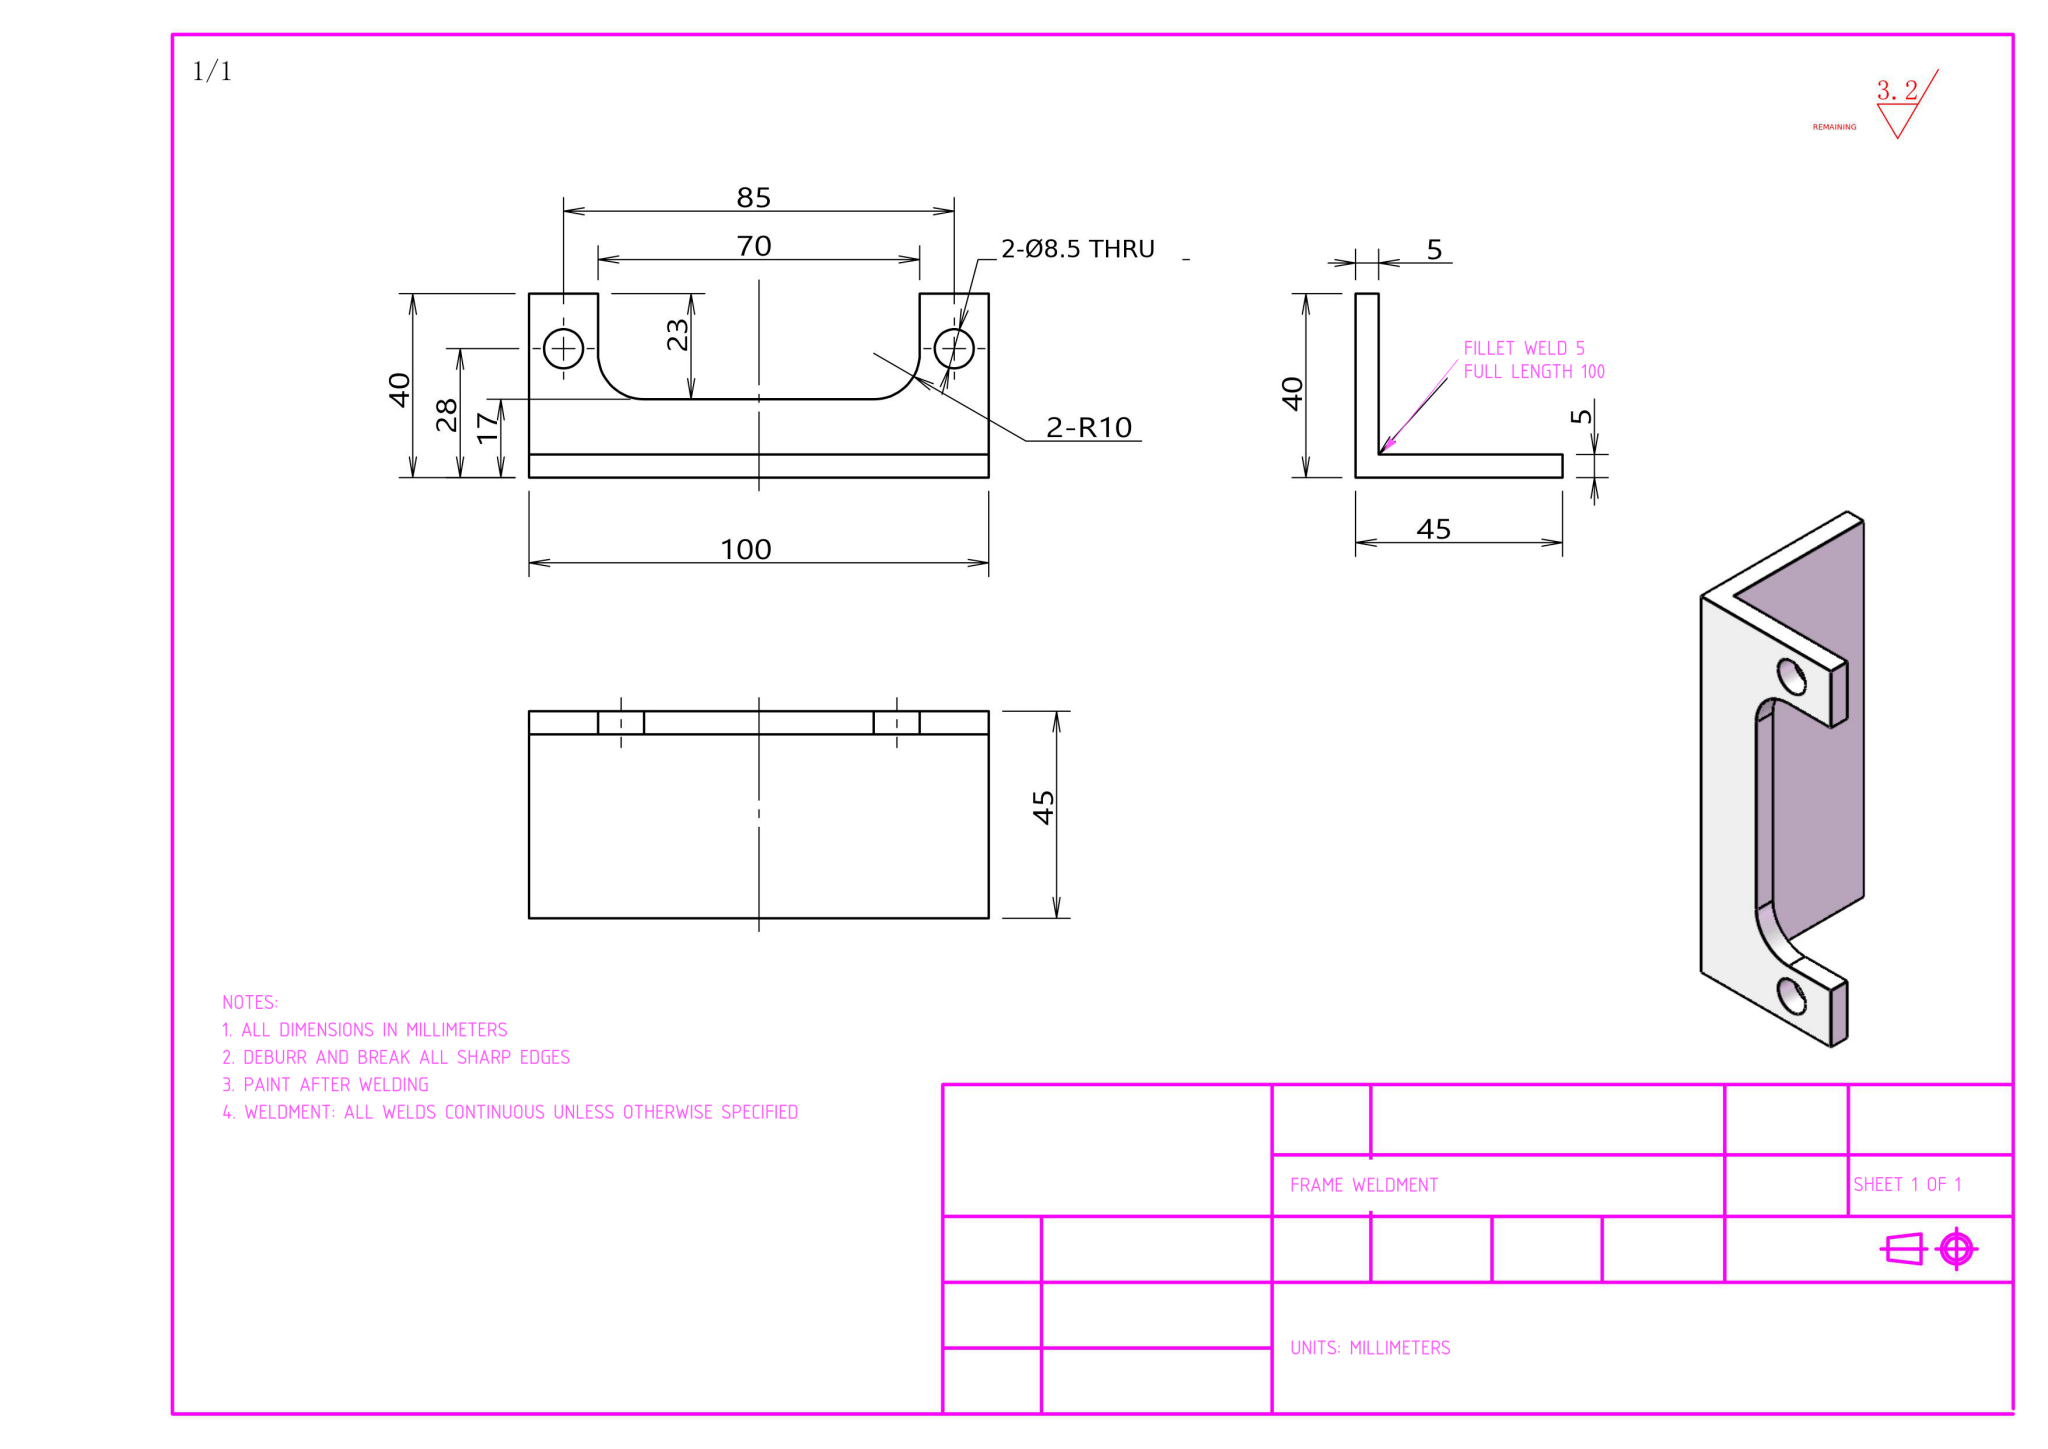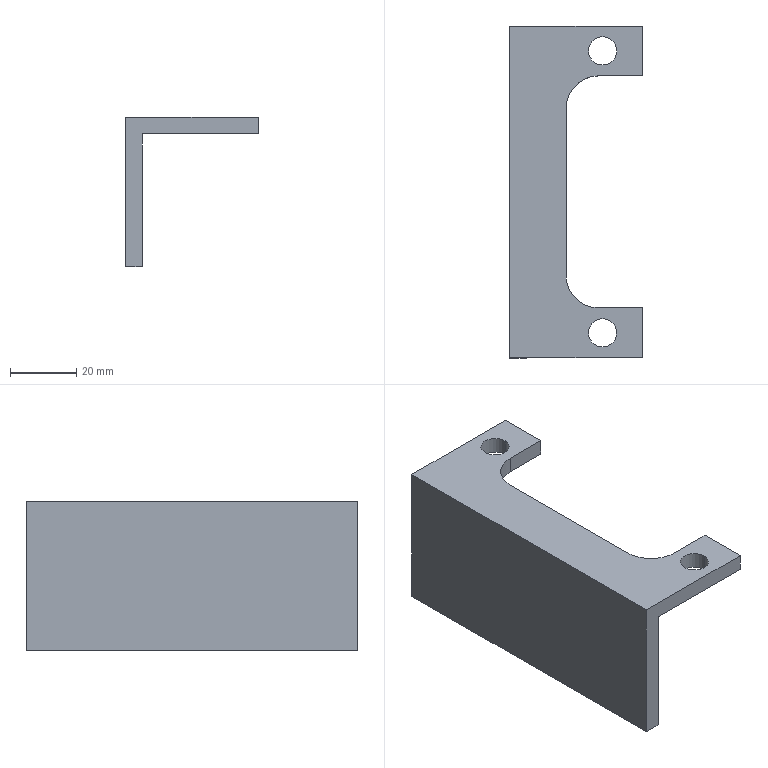Part | NX | mm | 1 solid | 18 faces | box 40 x 100 x 45 mm | volume 31597 mm3 | plane 12 | cylinder 6 | commonest cylinder face diameters 8.5 x4 20 x2
STEP:
#1=COLOUR_RGB('',1.,1.,1.);
#2=FILL_AREA_STYLE_COLOUR('',#1);
#3=FILL_AREA_STYLE('',(#2));
#4=SURFACE_STYLE_FILL_AREA(#3);
#5=SURFACE_SIDE_STYLE('',(#4));
#6=SURFACE_STYLE_USAGE(.BOTH.,#5);
#7=PRESENTATION_STYLE_ASSIGNMENT((#6));
#8=CARTESIAN_POINT('',(32.25,42.5,0.));
#9=VERTEX_POINT('',#8);
#10=CARTESIAN_POINT('',(23.75,42.5,0.));
#11=VERTEX_POINT('',#10);
#12=CARTESIAN_POINT('',(28.,42.5,0.));
#13=DIRECTION('',(0.,0.,-1.));
#14=DIRECTION('',(-1.,0.,0.));
#15=AXIS2_PLACEMENT_3D('',#12,#13,#14);
#16=CIRCLE('',#15,4.25);
#17=EDGE_CURVE('',#9,#11,#16,.T.);
#18=ORIENTED_EDGE('',*,*,#17,.F.);
#19=CARTESIAN_POINT('',(32.25,42.5,-5.));
#20=VERTEX_POINT('',#19);
#21=CARTESIAN_POINT('',(32.25,42.5,-5.));
#22=DIRECTION('',(0.,0.,-1.));
#23=VECTOR('',#22,1000.);
#24=LINE('',#21,#23);
#25=EDGE_CURVE('',#9,#20,#24,.T.);
#26=ORIENTED_EDGE('',*,*,#25,.T.);
#27=CARTESIAN_POINT('',(23.75,42.5,-5.));
#28=VERTEX_POINT('',#27);
#29=CARTESIAN_POINT('',(28.,42.5,-5.));
#30=DIRECTION('',(0.,0.,-1.));
#31=DIRECTION('',(-1.,0.,0.));
#32=AXIS2_PLACEMENT_3D('',#29,#30,#31);
#33=CIRCLE('',#32,4.25);
#34=EDGE_CURVE('',#20,#28,#33,.T.);
#35=ORIENTED_EDGE('',*,*,#34,.T.);
#36=CARTESIAN_POINT('',(23.75,42.5,-5.));
#37=DIRECTION('',(0.,0.,-1.));
#38=VECTOR('',#37,1000.);
#39=LINE('',#36,#38);
#40=EDGE_CURVE('',#11,#28,#39,.T.);
#41=ORIENTED_EDGE('',*,*,#40,.F.);
#42=EDGE_LOOP('',(#18,#26,#35,#41));
#43=FACE_OUTER_BOUND('',#42,.T.);
#44=CARTESIAN_POINT('',(28.,42.5,-5.));
#45=DIRECTION('',(0.,0.,-1.));
#46=DIRECTION('',(-1.,0.,0.));
#47=AXIS2_PLACEMENT_3D('',#44,#45,#46);
#48=CYLINDRICAL_SURFACE('',#47,4.25);
#49=ADVANCED_FACE('',(#43),#48,.F.);
#50=CARTESIAN_POINT('',(32.25,-42.5,0.));
#51=VERTEX_POINT('',#50);
#52=CARTESIAN_POINT('',(23.75,-42.5,0.));
#53=VERTEX_POINT('',#52);
#54=CARTESIAN_POINT('',(28.,-42.5,0.));
#55=DIRECTION('',(0.,0.,-1.));
#56=DIRECTION('',(-1.,0.,0.));
#57=AXIS2_PLACEMENT_3D('',#54,#55,#56);
#58=CIRCLE('',#57,4.25);
#59=EDGE_CURVE('',#51,#53,#58,.T.);
#60=ORIENTED_EDGE('',*,*,#59,.F.);
#61=CARTESIAN_POINT('',(32.25,-42.5,-5.));
#62=VERTEX_POINT('',#61);
#63=CARTESIAN_POINT('',(32.25,-42.5,-5.));
#64=DIRECTION('',(0.,0.,-1.));
#65=VECTOR('',#64,1000.);
#66=LINE('',#63,#65);
#67=EDGE_CURVE('',#51,#62,#66,.T.);
#68=ORIENTED_EDGE('',*,*,#67,.T.);
#69=CARTESIAN_POINT('',(23.75,-42.5,-5.));
#70=VERTEX_POINT('',#69);
#71=CARTESIAN_POINT('',(28.,-42.5,-5.));
#72=DIRECTION('',(0.,0.,-1.));
#73=DIRECTION('',(-1.,0.,0.));
#74=AXIS2_PLACEMENT_3D('',#71,#72,#73);
#75=CIRCLE('',#74,4.25);
#76=EDGE_CURVE('',#62,#70,#75,.T.);
#77=ORIENTED_EDGE('',*,*,#76,.T.);
#78=CARTESIAN_POINT('',(23.75,-42.5,-5.));
#79=DIRECTION('',(0.,0.,-1.));
#80=VECTOR('',#79,1000.);
#81=LINE('',#78,#80);
#82=EDGE_CURVE('',#53,#70,#81,.T.);
#83=ORIENTED_EDGE('',*,*,#82,.F.);
#84=EDGE_LOOP('',(#60,#68,#77,#83));
#85=FACE_OUTER_BOUND('',#84,.T.);
#86=CARTESIAN_POINT('',(28.,-42.5,-5.));
#87=DIRECTION('',(0.,0.,-1.));
#88=DIRECTION('',(-1.,0.,0.));
#89=AXIS2_PLACEMENT_3D('',#86,#87,#88);
#90=CYLINDRICAL_SURFACE('',#89,4.25);
#91=ADVANCED_FACE('',(#85),#90,.F.);
#92=CARTESIAN_POINT('',(40.,50.,-5.));
#93=VERTEX_POINT('',#92);
#94=CARTESIAN_POINT('',(40.,35.,-5.));
#95=VERTEX_POINT('',#94);
#96=CARTESIAN_POINT('',(40.,50.,-5.));
#97=DIRECTION('',(0.,-1.,0.));
#98=VECTOR('',#97,1000.);
#99=LINE('',#96,#98);
#100=EDGE_CURVE('',#93,#95,#99,.T.);
#101=ORIENTED_EDGE('',*,*,#100,.T.);
#102=CARTESIAN_POINT('',(27.,35.,-5.));
#103=VERTEX_POINT('',#102);
#104=CARTESIAN_POINT('',(40.,35.,-5.));
#105=DIRECTION('',(1.,-0.,-0.));
#106=VECTOR('',#105,1000.);
#107=LINE('',#104,#106);
#108=EDGE_CURVE('',#103,#95,#107,.T.);
#109=ORIENTED_EDGE('',*,*,#108,.F.);
#110=CARTESIAN_POINT('',(17.,25.,-5.));
#111=VERTEX_POINT('',#110);
#112=CARTESIAN_POINT('',(27.,25.,-5.));
#113=DIRECTION('',(0.,0.,1.));
#114=DIRECTION('',(1.,0.,-0.));
#115=AXIS2_PLACEMENT_3D('',#112,#113,#114);
#116=CIRCLE('',#115,10.);
#117=EDGE_CURVE('',#103,#111,#116,.T.);
#118=ORIENTED_EDGE('',*,*,#117,.T.);
#119=CARTESIAN_POINT('',(17.,-25.,-5.));
#120=VERTEX_POINT('',#119);
#121=CARTESIAN_POINT('',(17.,35.,-5.));
#122=DIRECTION('',(0.,1.,0.));
#123=VECTOR('',#122,1000.);
#124=LINE('',#121,#123);
#125=EDGE_CURVE('',#120,#111,#124,.T.);
#126=ORIENTED_EDGE('',*,*,#125,.F.);
#127=CARTESIAN_POINT('',(27.,-35.,-5.));
#128=VERTEX_POINT('',#127);
#129=CARTESIAN_POINT('',(27.,-25.,-5.));
#130=DIRECTION('',(0.,0.,1.));
#131=DIRECTION('',(1.,0.,-0.));
#132=AXIS2_PLACEMENT_3D('',#129,#130,#131);
#133=CIRCLE('',#132,10.);
#134=EDGE_CURVE('',#120,#128,#133,.T.);
#135=ORIENTED_EDGE('',*,*,#134,.T.);
#136=CARTESIAN_POINT('',(40.,-35.,-5.));
#137=VERTEX_POINT('',#136);
#138=CARTESIAN_POINT('',(40.,-35.,-5.));
#139=DIRECTION('',(-1.,0.,0.));
#140=VECTOR('',#139,1000.);
#141=LINE('',#138,#140);
#142=EDGE_CURVE('',#137,#128,#141,.T.);
#143=ORIENTED_EDGE('',*,*,#142,.F.);
#144=CARTESIAN_POINT('',(40.,-50.,-5.));
#145=VERTEX_POINT('',#144);
#146=CARTESIAN_POINT('',(40.,50.,-5.));
#147=DIRECTION('',(0.,-1.,0.));
#148=VECTOR('',#147,1000.);
#149=LINE('',#146,#148);
#150=EDGE_CURVE('',#137,#145,#149,.T.);
#151=ORIENTED_EDGE('',*,*,#150,.T.);
#152=CARTESIAN_POINT('',(5.,-50.,-5.));
#153=VERTEX_POINT('',#152);
#154=CARTESIAN_POINT('',(40.,-50.,-5.));
#155=DIRECTION('',(-1.,0.,0.));
#156=VECTOR('',#155,1000.);
#157=LINE('',#154,#156);
#158=EDGE_CURVE('',#145,#153,#157,.T.);
#159=ORIENTED_EDGE('',*,*,#158,.T.);
#160=CARTESIAN_POINT('',(5.,50.,-5.));
#161=VERTEX_POINT('',#160);
#162=CARTESIAN_POINT('',(5.,50.,-5.));
#163=DIRECTION('',(0.,-1.,0.));
#164=VECTOR('',#163,1000.);
#165=LINE('',#162,#164);
#166=EDGE_CURVE('',#161,#153,#165,.T.);
#167=ORIENTED_EDGE('',*,*,#166,.F.);
#168=CARTESIAN_POINT('',(40.,50.,-5.));
#169=DIRECTION('',(-1.,0.,0.));
#170=VECTOR('',#169,1000.);
#171=LINE('',#168,#170);
#172=EDGE_CURVE('',#93,#161,#171,.T.);
#173=ORIENTED_EDGE('',*,*,#172,.F.);
#174=EDGE_LOOP('',(#101,#109,#118,#126,#135,#143,#151,#159,#167,#173));
#175=FACE_OUTER_BOUND('',#174,.T.);
#176=CARTESIAN_POINT('',(28.,-42.5,-5.));
#177=DIRECTION('',(0.,0.,-1.));
#178=DIRECTION('',(-1.,0.,0.));
#179=AXIS2_PLACEMENT_3D('',#176,#177,#178);
#180=CIRCLE('',#179,4.25);
#181=EDGE_CURVE('',#70,#62,#180,.T.);
#182=ORIENTED_EDGE('',*,*,#181,.F.);
#183=ORIENTED_EDGE('',*,*,#76,.F.);
#184=EDGE_LOOP('',(#182,#183));
#185=FACE_BOUND('',#184,.T.);
#186=CARTESIAN_POINT('',(28.,42.5,-5.));
#187=DIRECTION('',(0.,0.,-1.));
#188=DIRECTION('',(-1.,0.,0.));
#189=AXIS2_PLACEMENT_3D('',#186,#187,#188);
#190=CIRCLE('',#189,4.25);
#191=EDGE_CURVE('',#28,#20,#190,.T.);
#192=ORIENTED_EDGE('',*,*,#191,.F.);
#193=ORIENTED_EDGE('',*,*,#34,.F.);
#194=EDGE_LOOP('',(#192,#193));
#195=FACE_BOUND('',#194,.T.);
#196=CARTESIAN_POINT('',(40.,50.,-5.));
#197=DIRECTION('',(0.,0.,1.));
#198=DIRECTION('',(1.,0.,-0.));
#199=AXIS2_PLACEMENT_3D('',#196,#197,#198);
#200=PLANE('',#199);
#201=ADVANCED_FACE('',(#175,#185,#195),#200,.F.);
#202=CARTESIAN_POINT('',(40.,50.,0.));
#203=VERTEX_POINT('',#202);
#204=CARTESIAN_POINT('',(40.,35.,0.));
#205=VERTEX_POINT('',#204);
#206=CARTESIAN_POINT('',(40.,50.,0.));
#207=DIRECTION('',(0.,-1.,0.));
#208=VECTOR('',#207,1000.);
#209=LINE('',#206,#208);
#210=EDGE_CURVE('',#203,#205,#209,.T.);
#211=ORIENTED_EDGE('',*,*,#210,.T.);
#212=CARTESIAN_POINT('',(40.,35.,0.));
#213=DIRECTION('',(-0.,0.,-1.));
#214=VECTOR('',#213,1000.);
#215=LINE('',#212,#214);
#216=EDGE_CURVE('',#205,#95,#215,.T.);
#217=ORIENTED_EDGE('',*,*,#216,.T.);
#218=ORIENTED_EDGE('',*,*,#100,.F.);
#219=CARTESIAN_POINT('',(40.,50.,0.));
#220=DIRECTION('',(0.,0.,-1.));
#221=VECTOR('',#220,1000.);
#222=LINE('',#219,#221);
#223=EDGE_CURVE('',#203,#93,#222,.T.);
#224=ORIENTED_EDGE('',*,*,#223,.F.);
#225=EDGE_LOOP('',(#211,#217,#218,#224));
#226=FACE_OUTER_BOUND('',#225,.T.);
#227=CARTESIAN_POINT('',(40.,50.,0.));
#228=DIRECTION('',(-1.,0.,0.));
#229=DIRECTION('',(0.,0.,1.));
#230=AXIS2_PLACEMENT_3D('',#227,#228,#229);
#231=PLANE('',#230);
#232=ADVANCED_FACE('',(#226),#231,.F.);
#233=CARTESIAN_POINT('',(28.,42.5,0.));
#234=DIRECTION('',(0.,0.,-1.));
#235=DIRECTION('',(-1.,0.,0.));
#236=AXIS2_PLACEMENT_3D('',#233,#234,#235);
#237=CIRCLE('',#236,4.25);
#238=EDGE_CURVE('',#11,#9,#237,.T.);
#239=ORIENTED_EDGE('',*,*,#238,.T.);
#240=ORIENTED_EDGE('',*,*,#17,.T.);
#241=EDGE_LOOP('',(#239,#240));
#242=FACE_BOUND('',#241,.T.);
#243=CARTESIAN_POINT('',(28.,-42.5,0.));
#244=DIRECTION('',(0.,0.,-1.));
#245=DIRECTION('',(-1.,0.,0.));
#246=AXIS2_PLACEMENT_3D('',#243,#244,#245);
#247=CIRCLE('',#246,4.25);
#248=EDGE_CURVE('',#53,#51,#247,.T.);
#249=ORIENTED_EDGE('',*,*,#248,.T.);
#250=ORIENTED_EDGE('',*,*,#59,.T.);
#251=EDGE_LOOP('',(#249,#250));
#252=FACE_BOUND('',#251,.T.);
#253=CARTESIAN_POINT('',(40.,-35.,0.));
#254=VERTEX_POINT('',#253);
#255=CARTESIAN_POINT('',(27.,-35.,0.));
#256=VERTEX_POINT('',#255);
#257=CARTESIAN_POINT('',(40.,-35.,0.));
#258=DIRECTION('',(-1.,0.,0.));
#259=VECTOR('',#258,1000.);
#260=LINE('',#257,#259);
#261=EDGE_CURVE('',#254,#256,#260,.T.);
#262=ORIENTED_EDGE('',*,*,#261,.T.);
#263=CARTESIAN_POINT('',(17.,-25.,0.));
#264=VERTEX_POINT('',#263);
#265=CARTESIAN_POINT('',(27.,-25.,0.));
#266=DIRECTION('',(0.,0.,-1.));
#267=DIRECTION('',(-1.,0.,0.));
#268=AXIS2_PLACEMENT_3D('',#265,#266,#267);
#269=CIRCLE('',#268,10.);
#270=EDGE_CURVE('',#256,#264,#269,.T.);
#271=ORIENTED_EDGE('',*,*,#270,.T.);
#272=CARTESIAN_POINT('',(17.,25.,0.));
#273=VERTEX_POINT('',#272);
#274=CARTESIAN_POINT('',(17.,35.,0.));
#275=DIRECTION('',(0.,1.,0.));
#276=VECTOR('',#275,1000.);
#277=LINE('',#274,#276);
#278=EDGE_CURVE('',#264,#273,#277,.T.);
#279=ORIENTED_EDGE('',*,*,#278,.T.);
#280=CARTESIAN_POINT('',(27.,35.,0.));
#281=VERTEX_POINT('',#280);
#282=CARTESIAN_POINT('',(27.,25.,0.));
#283=DIRECTION('',(0.,0.,-1.));
#284=DIRECTION('',(-1.,0.,0.));
#285=AXIS2_PLACEMENT_3D('',#282,#283,#284);
#286=CIRCLE('',#285,10.);
#287=EDGE_CURVE('',#273,#281,#286,.T.);
#288=ORIENTED_EDGE('',*,*,#287,.T.);
#289=CARTESIAN_POINT('',(40.,35.,0.));
#290=DIRECTION('',(1.,-0.,-0.));
#291=VECTOR('',#290,1000.);
#292=LINE('',#289,#291);
#293=EDGE_CURVE('',#281,#205,#292,.T.);
#294=ORIENTED_EDGE('',*,*,#293,.T.);
#295=ORIENTED_EDGE('',*,*,#210,.F.);
#296=CARTESIAN_POINT('',(0.,50.,0.));
#297=VERTEX_POINT('',#296);
#298=CARTESIAN_POINT('',(0.,50.,0.));
#299=DIRECTION('',(1.,0.,0.));
#300=VECTOR('',#299,1000.);
#301=LINE('',#298,#300);
#302=EDGE_CURVE('',#297,#203,#301,.T.);
#303=ORIENTED_EDGE('',*,*,#302,.F.);
#304=CARTESIAN_POINT('',(0.,-50.,0.));
#305=VERTEX_POINT('',#304);
#306=CARTESIAN_POINT('',(0.,50.,0.));
#307=DIRECTION('',(0.,-1.,0.));
#308=VECTOR('',#307,1000.);
#309=LINE('',#306,#308);
#310=EDGE_CURVE('',#297,#305,#309,.T.);
#311=ORIENTED_EDGE('',*,*,#310,.T.);
#312=CARTESIAN_POINT('',(40.,-50.,0.));
#313=VERTEX_POINT('',#312);
#314=CARTESIAN_POINT('',(0.,-50.,0.));
#315=DIRECTION('',(1.,0.,0.));
#316=VECTOR('',#315,1000.);
#317=LINE('',#314,#316);
#318=EDGE_CURVE('',#305,#313,#317,.T.);
#319=ORIENTED_EDGE('',*,*,#318,.T.);
#320=CARTESIAN_POINT('',(40.,50.,0.));
#321=DIRECTION('',(0.,-1.,0.));
#322=VECTOR('',#321,1000.);
#323=LINE('',#320,#322);
#324=EDGE_CURVE('',#254,#313,#323,.T.);
#325=ORIENTED_EDGE('',*,*,#324,.F.);
#326=EDGE_LOOP('',(#262,#271,#279,#288,#294,#295,#303,#311,#319,#325));
#327=FACE_OUTER_BOUND('',#326,.T.);
#328=CARTESIAN_POINT('',(0.,50.,0.));
#329=DIRECTION('',(0.,0.,-1.));
#330=DIRECTION('',(-1.,0.,0.));
#331=AXIS2_PLACEMENT_3D('',#328,#329,#330);
#332=PLANE('',#331);
#333=ADVANCED_FACE('',(#242,#252,#327),#332,.F.);
#334=ORIENTED_EDGE('',*,*,#150,.F.);
#335=CARTESIAN_POINT('',(40.,-35.,0.));
#336=DIRECTION('',(-0.,0.,-1.));
#337=VECTOR('',#336,1000.);
#338=LINE('',#335,#337);
#339=EDGE_CURVE('',#254,#137,#338,.T.);
#340=ORIENTED_EDGE('',*,*,#339,.F.);
#341=ORIENTED_EDGE('',*,*,#324,.T.);
#342=CARTESIAN_POINT('',(40.,-50.,0.));
#343=DIRECTION('',(0.,0.,-1.));
#344=VECTOR('',#343,1000.);
#345=LINE('',#342,#344);
#346=EDGE_CURVE('',#313,#145,#345,.T.);
#347=ORIENTED_EDGE('',*,*,#346,.T.);
#348=EDGE_LOOP('',(#334,#340,#341,#347));
#349=FACE_OUTER_BOUND('',#348,.T.);
#350=CARTESIAN_POINT('',(40.,50.,0.));
#351=DIRECTION('',(-1.,0.,0.));
#352=DIRECTION('',(0.,0.,1.));
#353=AXIS2_PLACEMENT_3D('',#350,#351,#352);
#354=PLANE('',#353);
#355=ADVANCED_FACE('',(#349),#354,.F.);
#356=CARTESIAN_POINT('',(5.,-50.,-45.));
#357=VERTEX_POINT('',#356);
#358=CARTESIAN_POINT('',(5.,-50.,-5.));
#359=DIRECTION('',(-0.,0.,-1.));
#360=VECTOR('',#359,1000.);
#361=LINE('',#358,#360);
#362=EDGE_CURVE('',#153,#357,#361,.T.);
#363=ORIENTED_EDGE('',*,*,#362,.T.);
#364=CARTESIAN_POINT('',(5.,50.,-45.));
#365=VERTEX_POINT('',#364);
#366=CARTESIAN_POINT('',(5.,50.,-45.));
#367=DIRECTION('',(0.,-1.,0.));
#368=VECTOR('',#367,1000.);
#369=LINE('',#366,#368);
#370=EDGE_CURVE('',#365,#357,#369,.T.);
#371=ORIENTED_EDGE('',*,*,#370,.F.);
#372=CARTESIAN_POINT('',(5.,50.,-5.));
#373=DIRECTION('',(-0.,0.,-1.));
#374=VECTOR('',#373,1000.);
#375=LINE('',#372,#374);
#376=EDGE_CURVE('',#161,#365,#375,.T.);
#377=ORIENTED_EDGE('',*,*,#376,.F.);
#378=ORIENTED_EDGE('',*,*,#166,.T.);
#379=EDGE_LOOP('',(#363,#371,#377,#378));
#380=FACE_OUTER_BOUND('',#379,.T.);
#381=CARTESIAN_POINT('',(5.,50.,-5.));
#382=DIRECTION('',(-1.,0.,0.));
#383=DIRECTION('',(0.,0.,1.));
#384=AXIS2_PLACEMENT_3D('',#381,#382,#383);
#385=PLANE('',#384);
#386=ADVANCED_FACE('',(#380),#385,.F.);
#387=CARTESIAN_POINT('',(-0.,-50.,-45.));
#388=VERTEX_POINT('',#387);
#389=CARTESIAN_POINT('',(5.,-50.,-45.));
#390=DIRECTION('',(-1.,0.,0.));
#391=VECTOR('',#390,1000.);
#392=LINE('',#389,#391);
#393=EDGE_CURVE('',#357,#388,#392,.T.);
#394=ORIENTED_EDGE('',*,*,#393,.T.);
#395=CARTESIAN_POINT('',(-0.,50.,-45.));
#396=VERTEX_POINT('',#395);
#397=CARTESIAN_POINT('',(-0.,50.,-45.));
#398=DIRECTION('',(0.,-1.,0.));
#399=VECTOR('',#398,1000.);
#400=LINE('',#397,#399);
#401=EDGE_CURVE('',#396,#388,#400,.T.);
#402=ORIENTED_EDGE('',*,*,#401,.F.);
#403=CARTESIAN_POINT('',(5.,50.,-45.));
#404=DIRECTION('',(-1.,0.,0.));
#405=VECTOR('',#404,1000.);
#406=LINE('',#403,#405);
#407=EDGE_CURVE('',#365,#396,#406,.T.);
#408=ORIENTED_EDGE('',*,*,#407,.F.);
#409=ORIENTED_EDGE('',*,*,#370,.T.);
#410=EDGE_LOOP('',(#394,#402,#408,#409));
#411=FACE_OUTER_BOUND('',#410,.T.);
#412=CARTESIAN_POINT('',(5.,50.,-45.));
#413=DIRECTION('',(0.,0.,1.));
#414=DIRECTION('',(1.,0.,0.));
#415=AXIS2_PLACEMENT_3D('',#412,#413,#414);
#416=PLANE('',#415);
#417=ADVANCED_FACE('',(#411),#416,.F.);
#418=CARTESIAN_POINT('',(-0.,-50.,-45.));
#419=DIRECTION('',(0.,0.,1.));
#420=VECTOR('',#419,1000.);
#421=LINE('',#418,#420);
#422=EDGE_CURVE('',#388,#305,#421,.T.);
#423=ORIENTED_EDGE('',*,*,#422,.T.);
#424=ORIENTED_EDGE('',*,*,#310,.F.);
#425=CARTESIAN_POINT('',(-0.,50.,-45.));
#426=DIRECTION('',(0.,0.,1.));
#427=VECTOR('',#426,1000.);
#428=LINE('',#425,#427);
#429=EDGE_CURVE('',#396,#297,#428,.T.);
#430=ORIENTED_EDGE('',*,*,#429,.F.);
#431=ORIENTED_EDGE('',*,*,#401,.T.);
#432=EDGE_LOOP('',(#423,#424,#430,#431));
#433=FACE_OUTER_BOUND('',#432,.T.);
#434=CARTESIAN_POINT('',(-0.,50.,-45.));
#435=DIRECTION('',(1.,0.,-0.));
#436=DIRECTION('',(-0.,0.,-1.));
#437=AXIS2_PLACEMENT_3D('',#434,#435,#436);
#438=PLANE('',#437);
#439=ADVANCED_FACE('',(#433),#438,.F.);
#440=ORIENTED_EDGE('',*,*,#302,.T.);
#441=ORIENTED_EDGE('',*,*,#223,.T.);
#442=ORIENTED_EDGE('',*,*,#172,.T.);
#443=ORIENTED_EDGE('',*,*,#376,.T.);
#444=ORIENTED_EDGE('',*,*,#407,.T.);
#445=ORIENTED_EDGE('',*,*,#429,.T.);
#446=EDGE_LOOP('',(#440,#441,#442,#443,#444,#445));
#447=FACE_OUTER_BOUND('',#446,.T.);
#448=CARTESIAN_POINT('',(0.,50.,0.));
#449=DIRECTION('',(0.,1.,0.));
#450=DIRECTION('',(0.,0.,1.));
#451=AXIS2_PLACEMENT_3D('',#448,#449,#450);
#452=PLANE('',#451);
#453=ADVANCED_FACE('',(#447),#452,.T.);
#454=ORIENTED_EDGE('',*,*,#318,.F.);
#455=ORIENTED_EDGE('',*,*,#422,.F.);
#456=ORIENTED_EDGE('',*,*,#393,.F.);
#457=ORIENTED_EDGE('',*,*,#362,.F.);
#458=ORIENTED_EDGE('',*,*,#158,.F.);
#459=ORIENTED_EDGE('',*,*,#346,.F.);
#460=EDGE_LOOP('',(#454,#455,#456,#457,#458,#459));
#461=FACE_OUTER_BOUND('',#460,.T.);
#462=CARTESIAN_POINT('',(0.,-50.,0.));
#463=DIRECTION('',(0.,1.,0.));
#464=DIRECTION('',(0.,0.,1.));
#465=AXIS2_PLACEMENT_3D('',#462,#463,#464);
#466=PLANE('',#465);
#467=ADVANCED_FACE('',(#461),#466,.F.);
#468=ORIENTED_EDGE('',*,*,#293,.F.);
#469=CARTESIAN_POINT('',(27.,35.,-5.));
#470=DIRECTION('',(-0.,0.,-1.));
#471=VECTOR('',#470,1000.);
#472=LINE('',#469,#471);
#473=EDGE_CURVE('',#281,#103,#472,.T.);
#474=ORIENTED_EDGE('',*,*,#473,.T.);
#475=ORIENTED_EDGE('',*,*,#108,.T.);
#476=ORIENTED_EDGE('',*,*,#216,.F.);
#477=EDGE_LOOP('',(#468,#474,#475,#476));
#478=FACE_OUTER_BOUND('',#477,.T.);
#479=CARTESIAN_POINT('',(40.,35.,0.));
#480=DIRECTION('',(0.,1.,-0.));
#481=DIRECTION('',(-1.,0.,0.));
#482=AXIS2_PLACEMENT_3D('',#479,#480,#481);
#483=PLANE('',#482);
#484=ADVANCED_FACE('',(#478),#483,.F.);
#485=ORIENTED_EDGE('',*,*,#278,.F.);
#486=CARTESIAN_POINT('',(17.,-25.,-5.));
#487=DIRECTION('',(-0.,0.,-1.));
#488=VECTOR('',#487,1000.);
#489=LINE('',#486,#488);
#490=EDGE_CURVE('',#264,#120,#489,.T.);
#491=ORIENTED_EDGE('',*,*,#490,.T.);
#492=ORIENTED_EDGE('',*,*,#125,.T.);
#493=CARTESIAN_POINT('',(17.,25.,0.));
#494=DIRECTION('',(0.,0.,1.));
#495=VECTOR('',#494,1000.);
#496=LINE('',#493,#495);
#497=EDGE_CURVE('',#111,#273,#496,.T.);
#498=ORIENTED_EDGE('',*,*,#497,.T.);
#499=EDGE_LOOP('',(#485,#491,#492,#498));
#500=FACE_OUTER_BOUND('',#499,.T.);
#501=CARTESIAN_POINT('',(17.,35.,0.));
#502=DIRECTION('',(-1.,0.,0.));
#503=DIRECTION('',(-0.,-1.,0.));
#504=AXIS2_PLACEMENT_3D('',#501,#502,#503);
#505=PLANE('',#504);
#506=ADVANCED_FACE('',(#500),#505,.F.);
#507=ORIENTED_EDGE('',*,*,#142,.T.);
#508=CARTESIAN_POINT('',(27.,-35.,0.));
#509=DIRECTION('',(0.,0.,1.));
#510=VECTOR('',#509,1000.);
#511=LINE('',#508,#510);
#512=EDGE_CURVE('',#128,#256,#511,.T.);
#513=ORIENTED_EDGE('',*,*,#512,.T.);
#514=ORIENTED_EDGE('',*,*,#261,.F.);
#515=ORIENTED_EDGE('',*,*,#339,.T.);
#516=EDGE_LOOP('',(#507,#513,#514,#515));
#517=FACE_OUTER_BOUND('',#516,.T.);
#518=CARTESIAN_POINT('',(40.,-35.,0.));
#519=DIRECTION('',(0.,-1.,0.));
#520=DIRECTION('',(0.,0.,-1.));
#521=AXIS2_PLACEMENT_3D('',#518,#519,#520);
#522=PLANE('',#521);
#523=ADVANCED_FACE('',(#517),#522,.F.);
#524=ORIENTED_EDGE('',*,*,#270,.F.);
#525=ORIENTED_EDGE('',*,*,#512,.F.);
#526=ORIENTED_EDGE('',*,*,#134,.F.);
#527=ORIENTED_EDGE('',*,*,#490,.F.);
#528=EDGE_LOOP('',(#524,#525,#526,#527));
#529=FACE_OUTER_BOUND('',#528,.T.);
#530=CARTESIAN_POINT('',(27.,-25.,0.));
#531=DIRECTION('',(0.,0.,1.));
#532=DIRECTION('',(1.,0.,-0.));
#533=AXIS2_PLACEMENT_3D('',#530,#531,#532);
#534=CYLINDRICAL_SURFACE('',#533,10.);
#535=ADVANCED_FACE('',(#529),#534,.F.);
#536=ORIENTED_EDGE('',*,*,#287,.F.);
#537=ORIENTED_EDGE('',*,*,#497,.F.);
#538=ORIENTED_EDGE('',*,*,#117,.F.);
#539=ORIENTED_EDGE('',*,*,#473,.F.);
#540=EDGE_LOOP('',(#536,#537,#538,#539));
#541=FACE_OUTER_BOUND('',#540,.T.);
#542=CARTESIAN_POINT('',(27.,25.,0.));
#543=DIRECTION('',(0.,0.,1.));
#544=DIRECTION('',(1.,0.,-0.));
#545=AXIS2_PLACEMENT_3D('',#542,#543,#544);
#546=CYLINDRICAL_SURFACE('',#545,10.);
#547=ADVANCED_FACE('',(#541),#546,.F.);
#548=ORIENTED_EDGE('',*,*,#67,.F.);
#549=ORIENTED_EDGE('',*,*,#248,.F.);
#550=ORIENTED_EDGE('',*,*,#82,.T.);
#551=ORIENTED_EDGE('',*,*,#181,.T.);
#552=EDGE_LOOP('',(#548,#549,#550,#551));
#553=FACE_OUTER_BOUND('',#552,.T.);
#554=CARTESIAN_POINT('',(28.,-42.5,-5.));
#555=DIRECTION('',(0.,0.,-1.));
#556=DIRECTION('',(-1.,0.,0.));
#557=AXIS2_PLACEMENT_3D('',#554,#555,#556);
#558=CYLINDRICAL_SURFACE('',#557,4.25);
#559=ADVANCED_FACE('',(#553),#558,.F.);
#560=ORIENTED_EDGE('',*,*,#25,.F.);
#561=ORIENTED_EDGE('',*,*,#238,.F.);
#562=ORIENTED_EDGE('',*,*,#40,.T.);
#563=ORIENTED_EDGE('',*,*,#191,.T.);
#564=EDGE_LOOP('',(#560,#561,#562,#563));
#565=FACE_OUTER_BOUND('',#564,.T.);
#566=CARTESIAN_POINT('',(28.,42.5,-5.));
#567=DIRECTION('',(0.,0.,-1.));
#568=DIRECTION('',(-1.,0.,0.));
#569=AXIS2_PLACEMENT_3D('',#566,#567,#568);
#570=CYLINDRICAL_SURFACE('',#569,4.25);
#571=ADVANCED_FACE('',(#565),#570,.F.);
#572=CLOSED_SHELL('',(#49,#91,#201,#232,#333,#355,#386,#417,#439,#453,#467,#484,#506,#523,#535,#547,#559,#571));
#573=MANIFOLD_SOLID_BREP('',#572);
#574=CARTESIAN_POINT('',(0.,0.,0.));
#575=DIRECTION('',(0.,0.,1.));
#576=DIRECTION('',(1.,0.,0.));
#577=AXIS2_PLACEMENT_3D('',#574,#575,#576);
#578=(LENGTH_UNIT()NAMED_UNIT(*)SI_UNIT(.MILLI.,.METRE.));
#579=UNCERTAINTY_MEASURE_WITH_UNIT(LENGTH_MEASURE(0.00001),#578,'','');
#580=(NAMED_UNIT(*)PLANE_ANGLE_UNIT()SI_UNIT($,.RADIAN.));
#581=(NAMED_UNIT(*)SI_UNIT($,.STERADIAN.)SOLID_ANGLE_UNIT());
#582=(GEOMETRIC_REPRESENTATION_CONTEXT(3)GLOBAL_UNCERTAINTY_ASSIGNED_CONTEXT((#579))GLOBAL_UNIT_ASSIGNED_CONTEXT((#578,#580,#581))REPRESENTATION_CONTEXT('',''));
#583=ADVANCED_BREP_SHAPE_REPRESENTATION('',(#573,#577),#582);
#584=STYLED_ITEM('',(#7),#583);
#585=PRESENTATION_LAYER_ASSIGNMENT('','',(#584));
#586=COLOUR_RGB('',1.,1.,1.);
#587=FILL_AREA_STYLE_COLOUR('',#586);
#588=FILL_AREA_STYLE('',(#587));
#589=SURFACE_STYLE_FILL_AREA(#588);
#590=SURFACE_SIDE_STYLE('',(#589));
#591=SURFACE_STYLE_USAGE(.BOTH.,#590);
#592=PRESENTATION_STYLE_ASSIGNMENT((#591));
#593=STYLED_ITEM('',(#592),#573);
#594=PRESENTATION_LAYER_ASSIGNMENT('','',(#593));
#595=(LENGTH_UNIT()NAMED_UNIT(*)SI_UNIT(.MILLI.,.METRE.));
#596=UNCERTAINTY_MEASURE_WITH_UNIT(LENGTH_MEASURE(0.00001),#595,'','');
#597=(NAMED_UNIT(*)PLANE_ANGLE_UNIT()SI_UNIT($,.RADIAN.));
#598=(NAMED_UNIT(*)SI_UNIT($,.STERADIAN.)SOLID_ANGLE_UNIT());
#599=(GEOMETRIC_REPRESENTATION_CONTEXT(3)GLOBAL_UNCERTAINTY_ASSIGNED_CONTEXT((#596))GLOBAL_UNIT_ASSIGNED_CONTEXT((#595,#597,#598))REPRESENTATION_CONTEXT('',''));
#600=MECHANICAL_DESIGN_GEOMETRIC_PRESENTATION_REPRESENTATION('',(#593),#599);
#601=(LENGTH_UNIT()NAMED_UNIT(*)SI_UNIT(.MILLI.,.METRE.));
#602=UNCERTAINTY_MEASURE_WITH_UNIT(LENGTH_MEASURE(0.00001),#601,'','');
#603=(NAMED_UNIT(*)PLANE_ANGLE_UNIT()SI_UNIT($,.RADIAN.));
#604=(NAMED_UNIT(*)SI_UNIT($,.STERADIAN.)SOLID_ANGLE_UNIT());
#605=(GEOMETRIC_REPRESENTATION_CONTEXT(3)GLOBAL_UNCERTAINTY_ASSIGNED_CONTEXT((#602))GLOBAL_UNIT_ASSIGNED_CONTEXT((#601,#603,#604))REPRESENTATION_CONTEXT('',''));
#606=MECHANICAL_DESIGN_GEOMETRIC_PRESENTATION_REPRESENTATION('',(#584),#605);